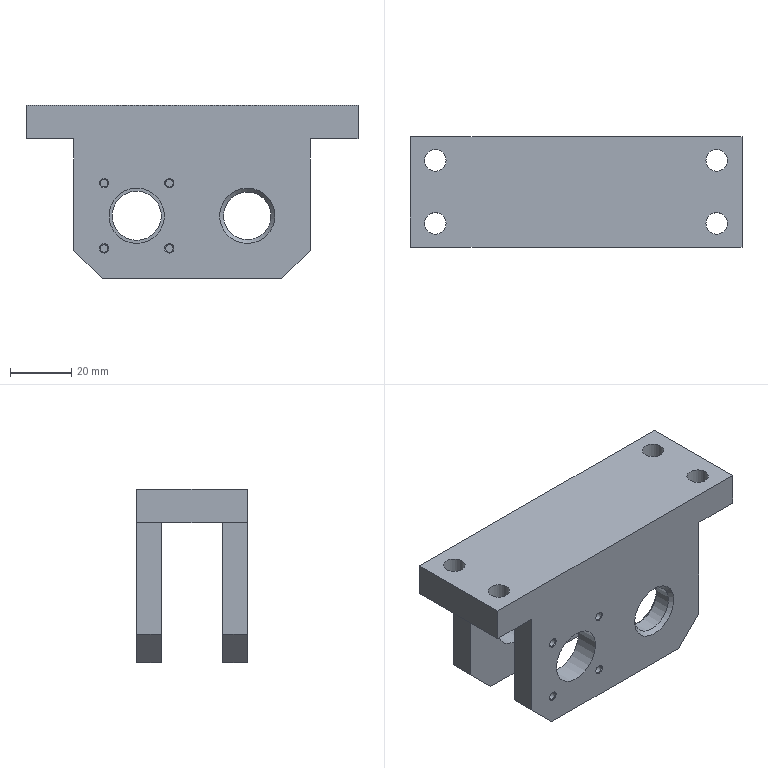Component | NX | CLHKJG_01_GEAR_SUPPORT | 1 solid | 60 faces | volume 87185 mm3 | plane 22 | cylinder 20 | cone 18 | commonest cylinder face diameters 2.5 x8 7 x4 10 x4 18 x2 15.5 x1 16 x1